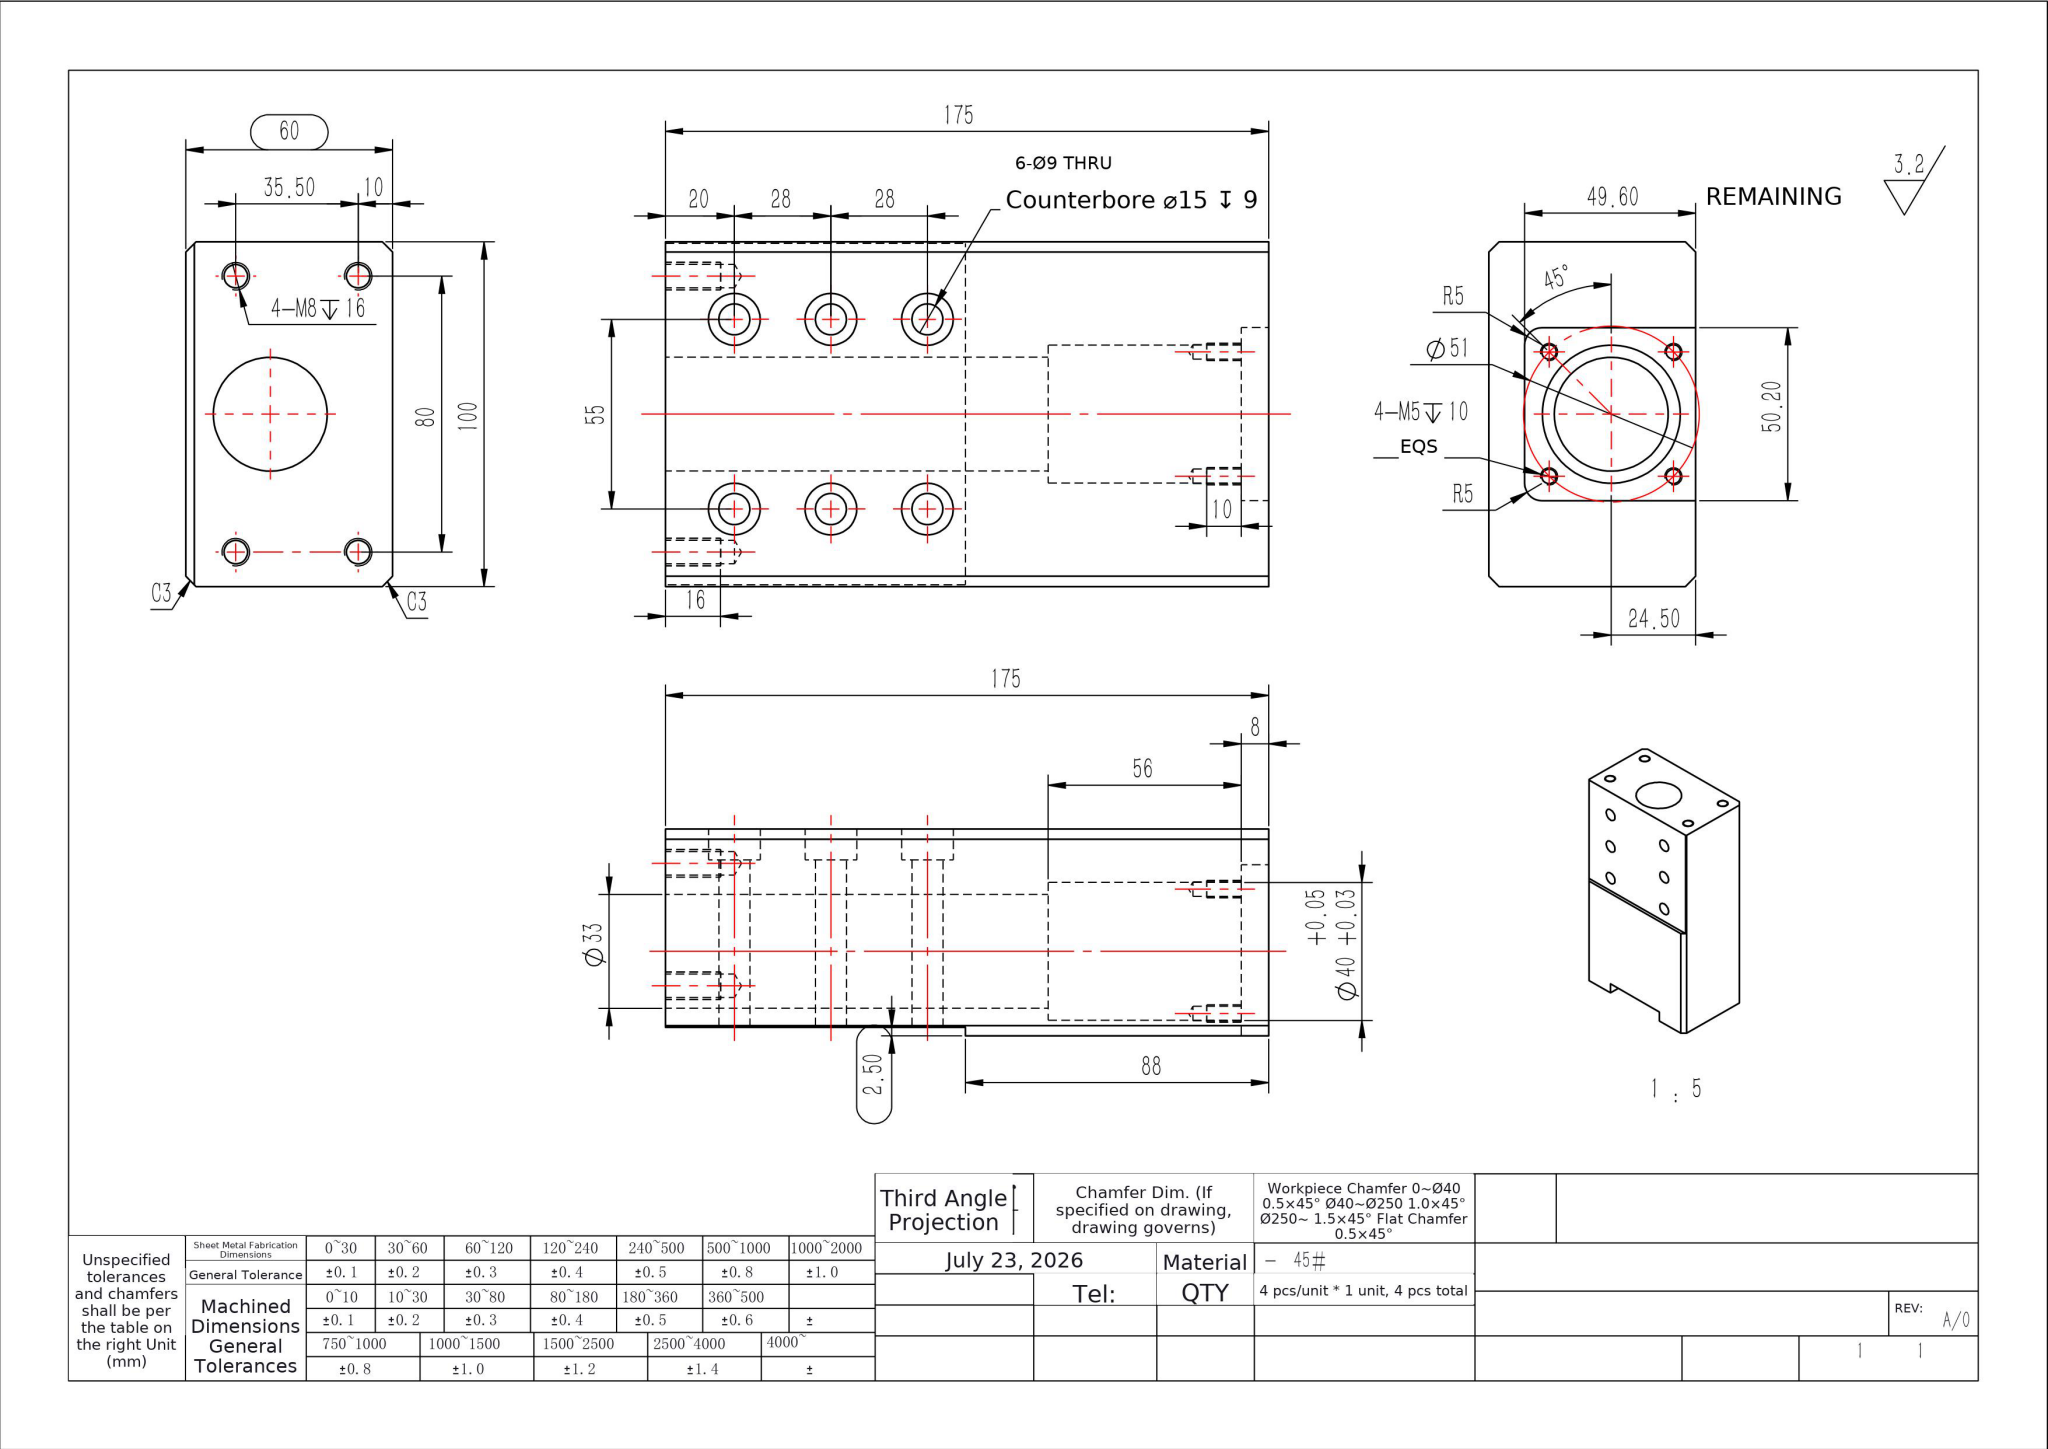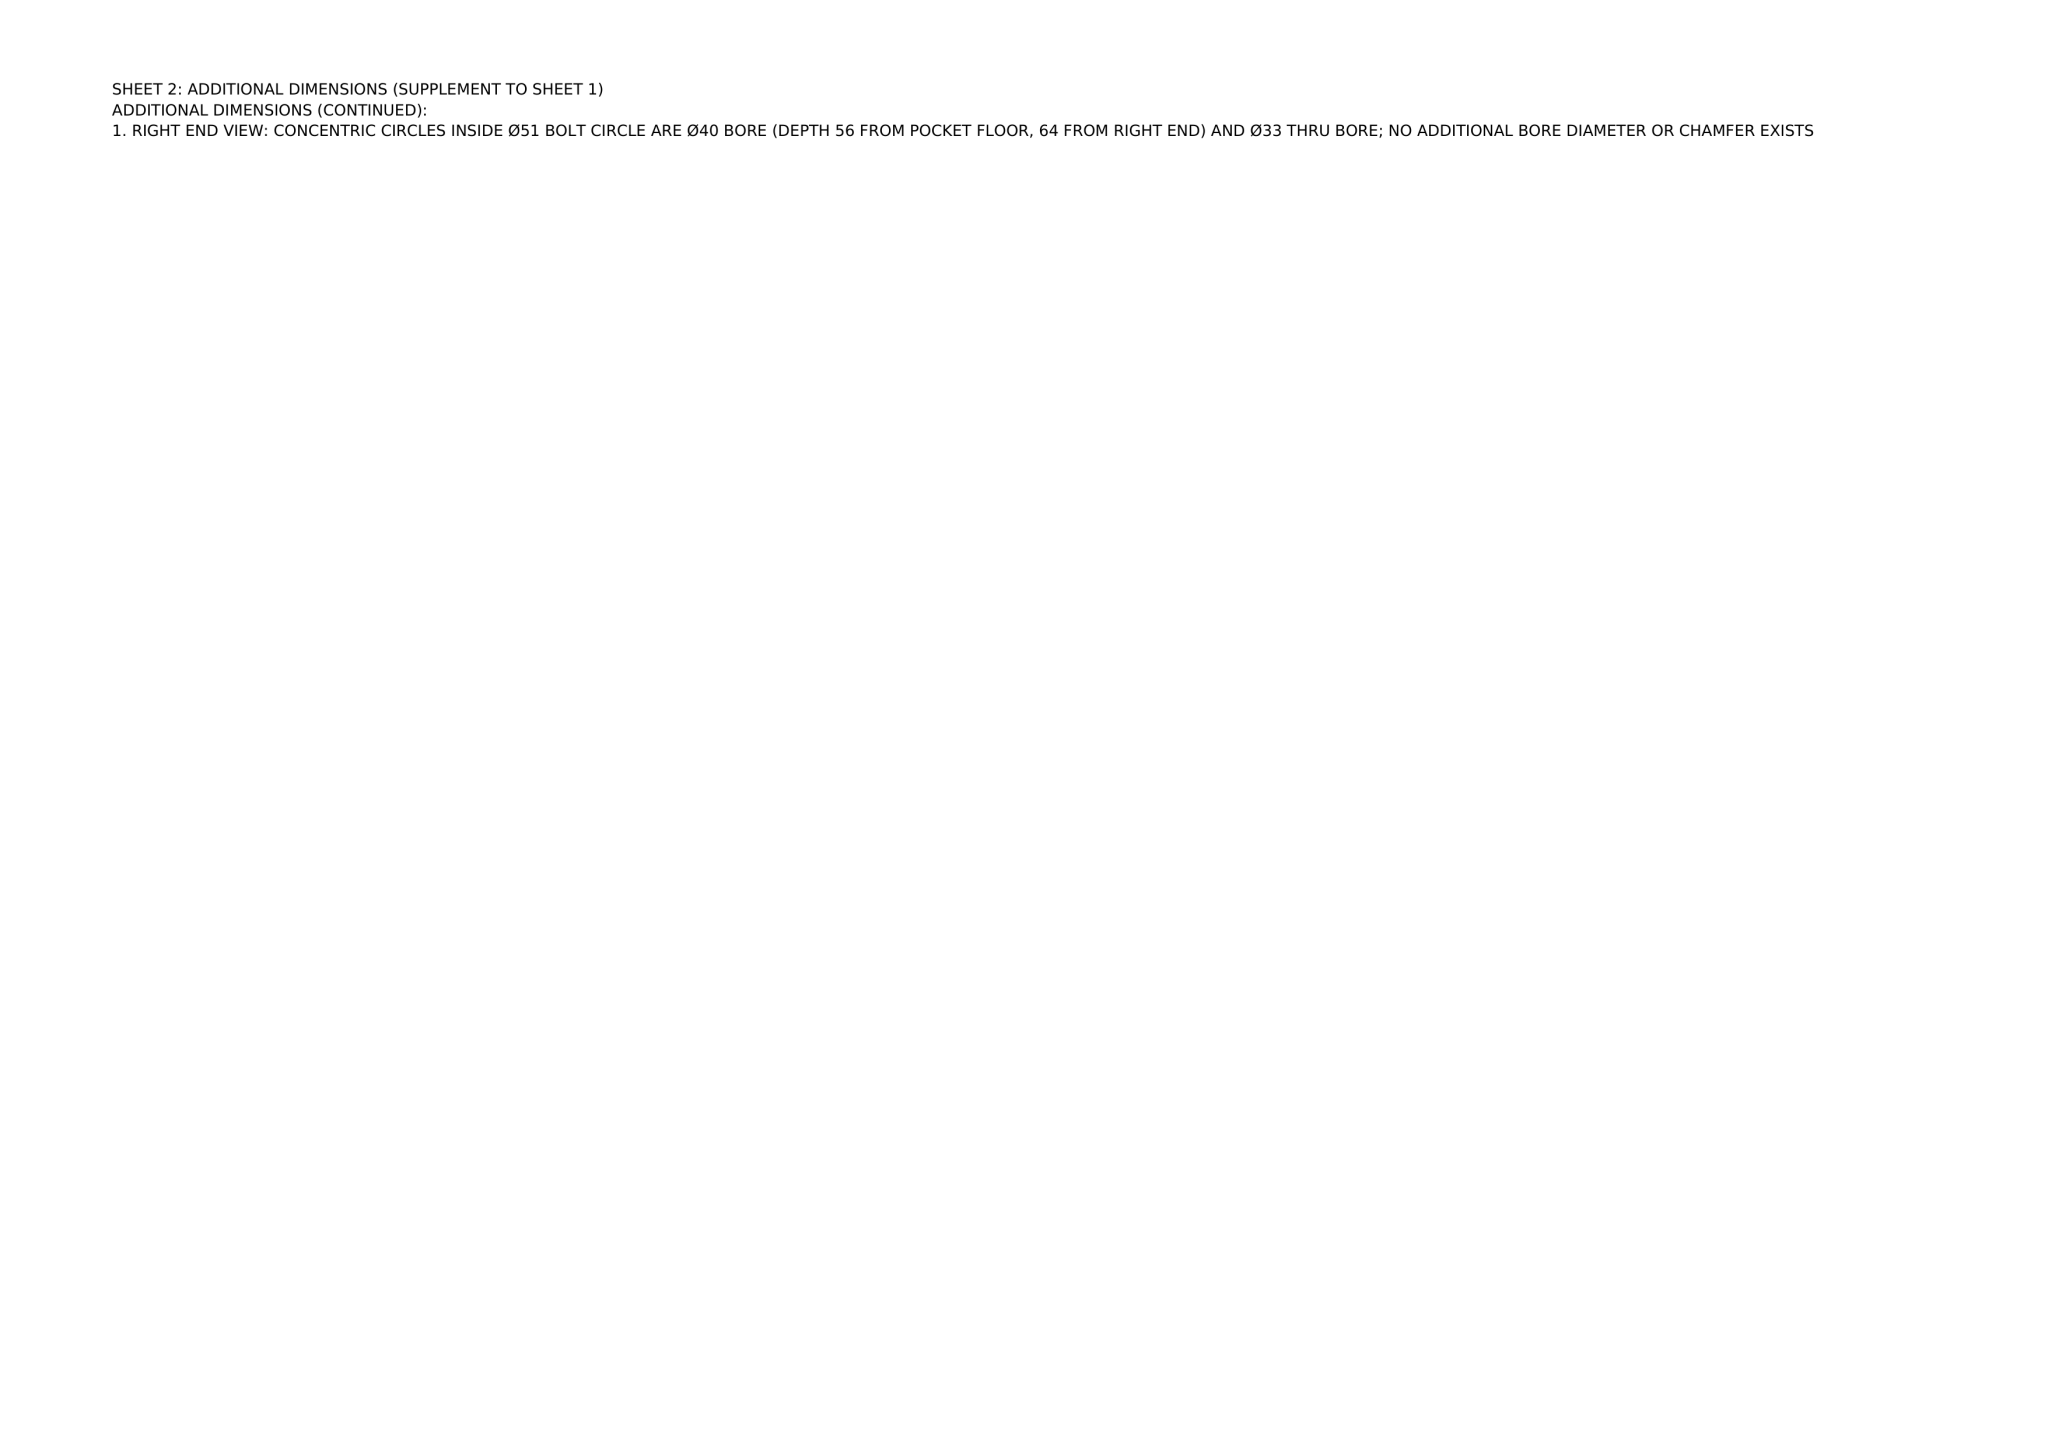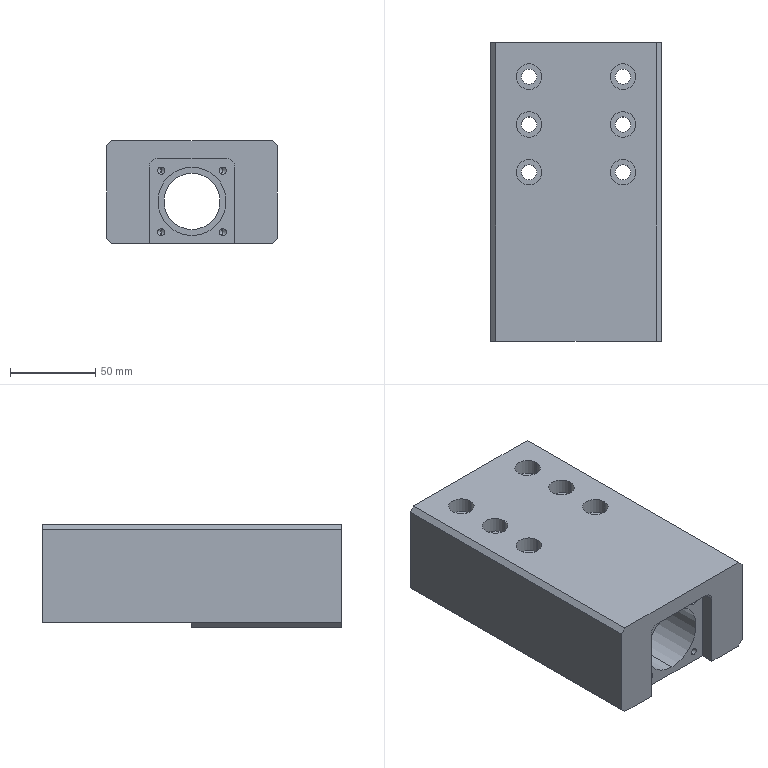Part | NX | mm | 1 solid | 85 faces | box 100 x 175 x 60 mm | volume 808859 mm3 | cylinder 46 | plane 23 | cone 16 | commonest cylinder face diameters 15 x12 9 x12 4.2 x8 6.8 x8 40 x2 33 x2 10 x2